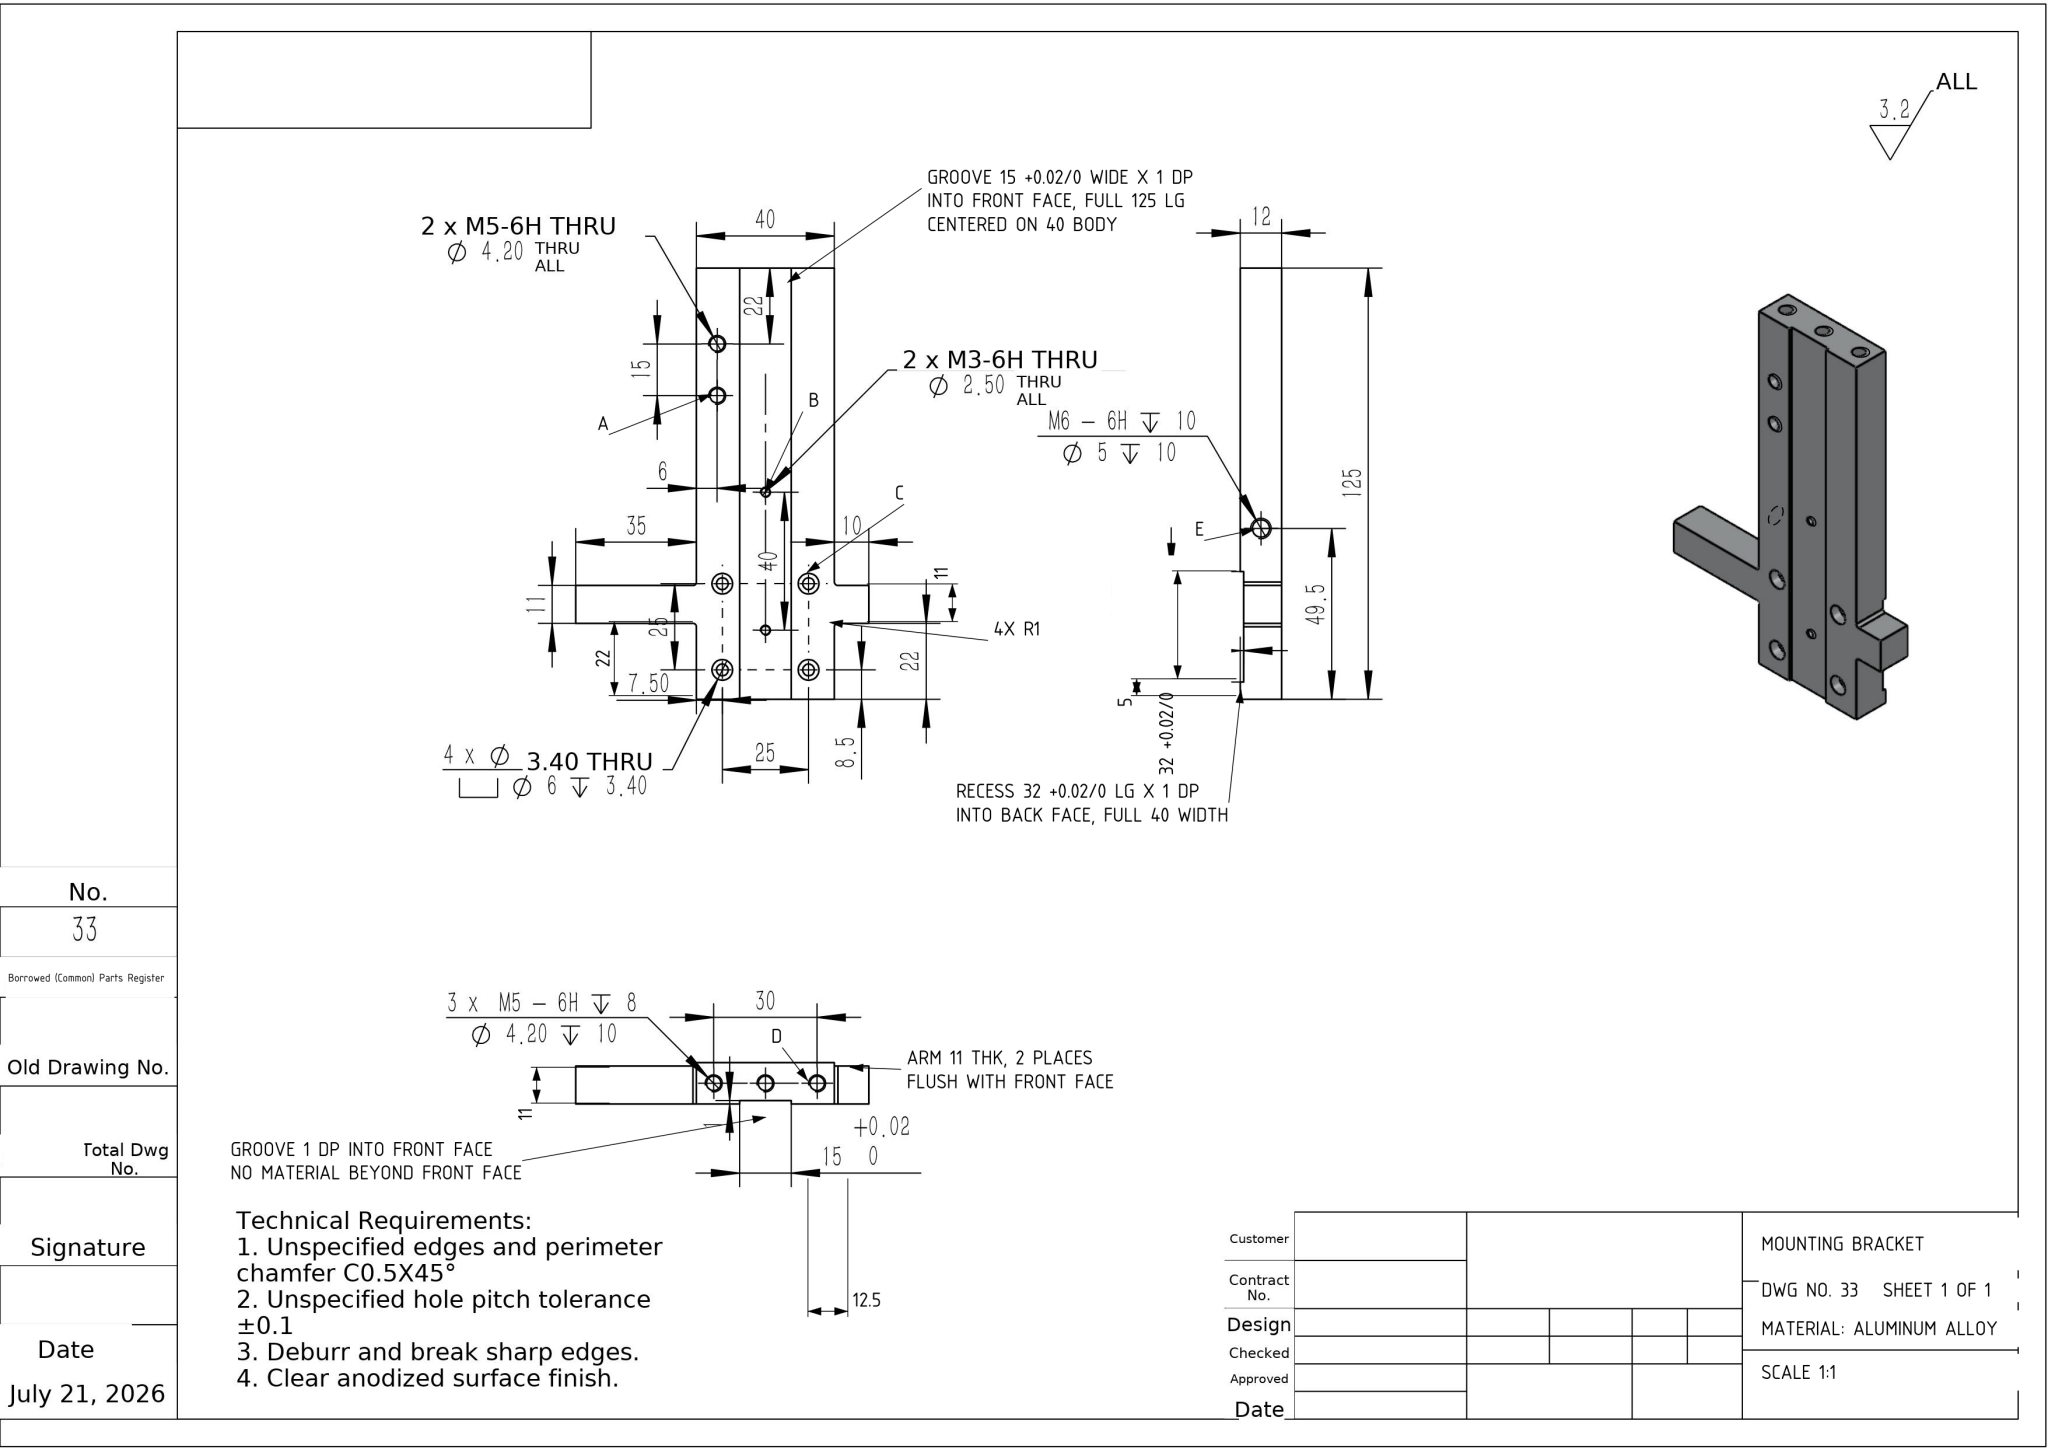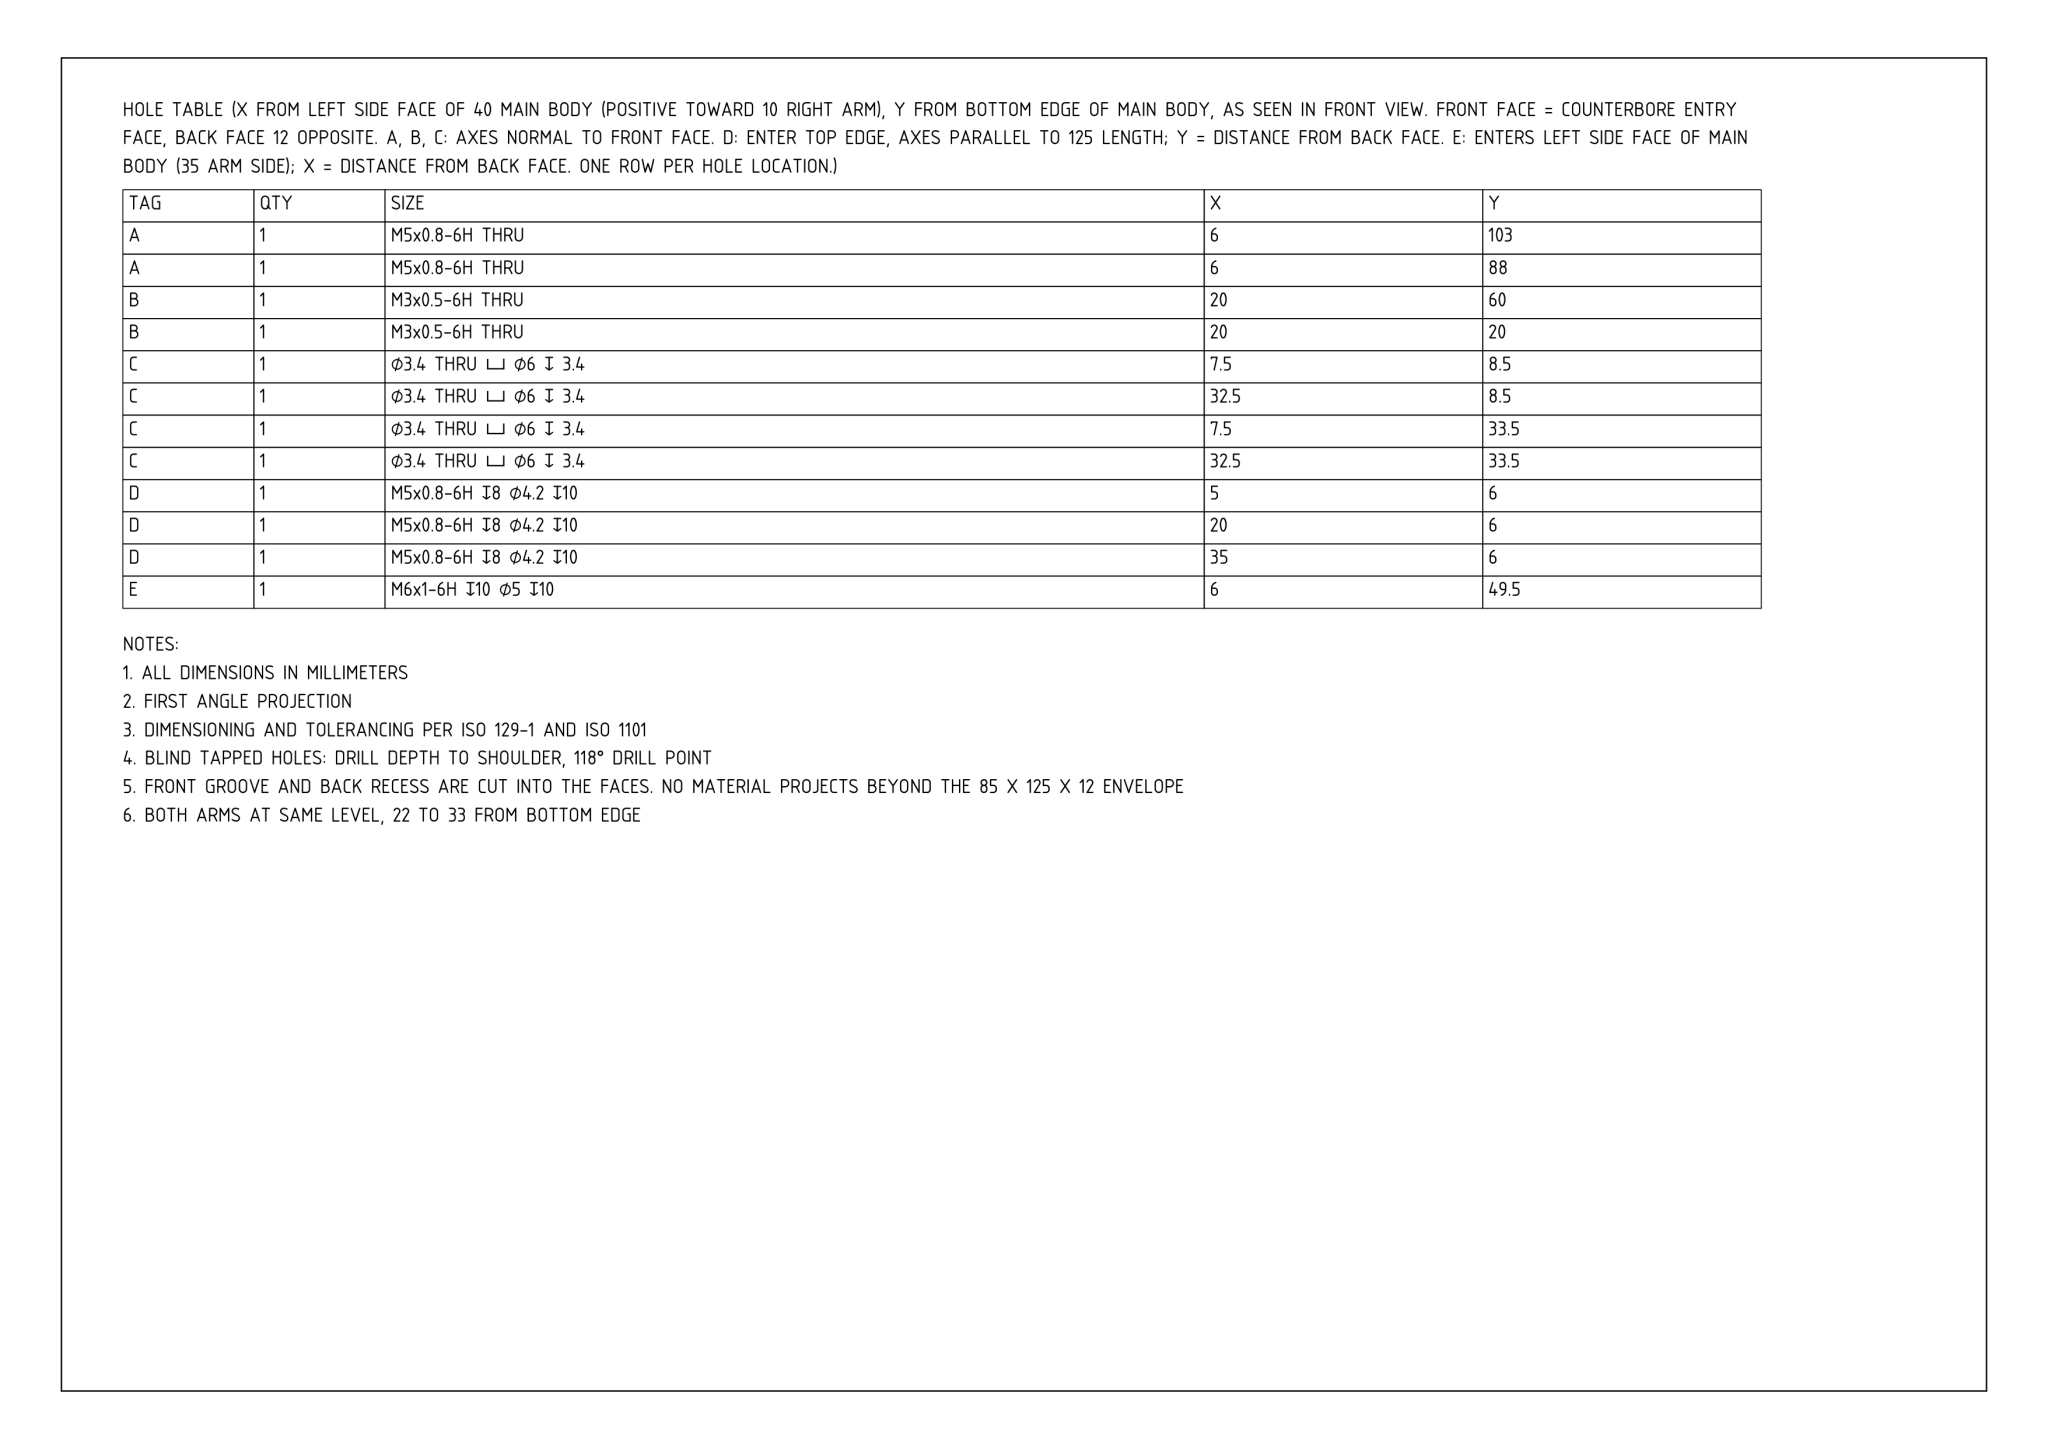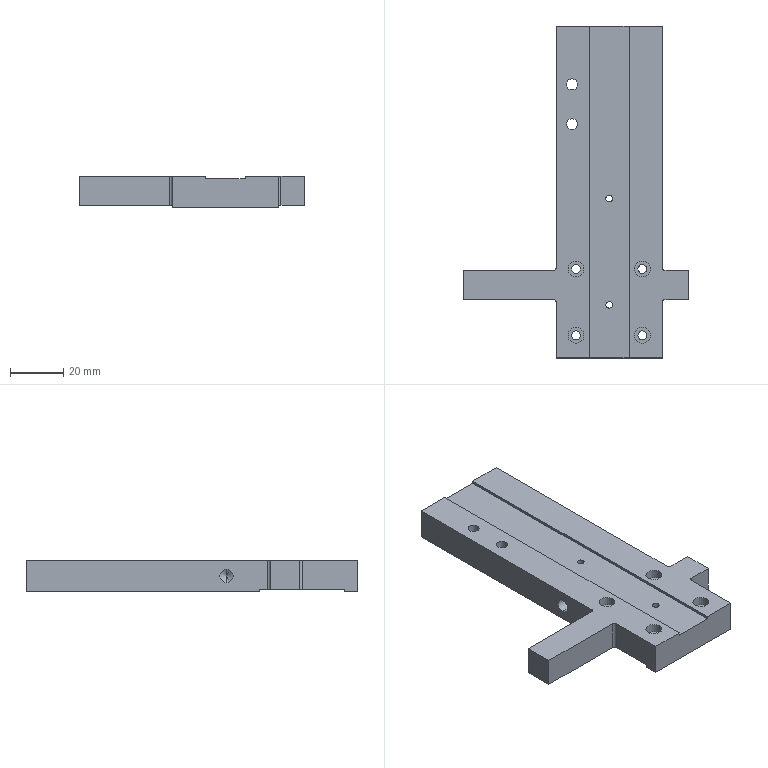Part | NX | mm | 1 solid | 70 faces | box 85 x 125 x 12 mm | volume 60564 mm3 | cylinder 36 | plane 26 | cone 8 | commonest cylinder face diameters 4.2 x10 6 x8 3.4 x8 2.5 x4 2 x4 5 x2